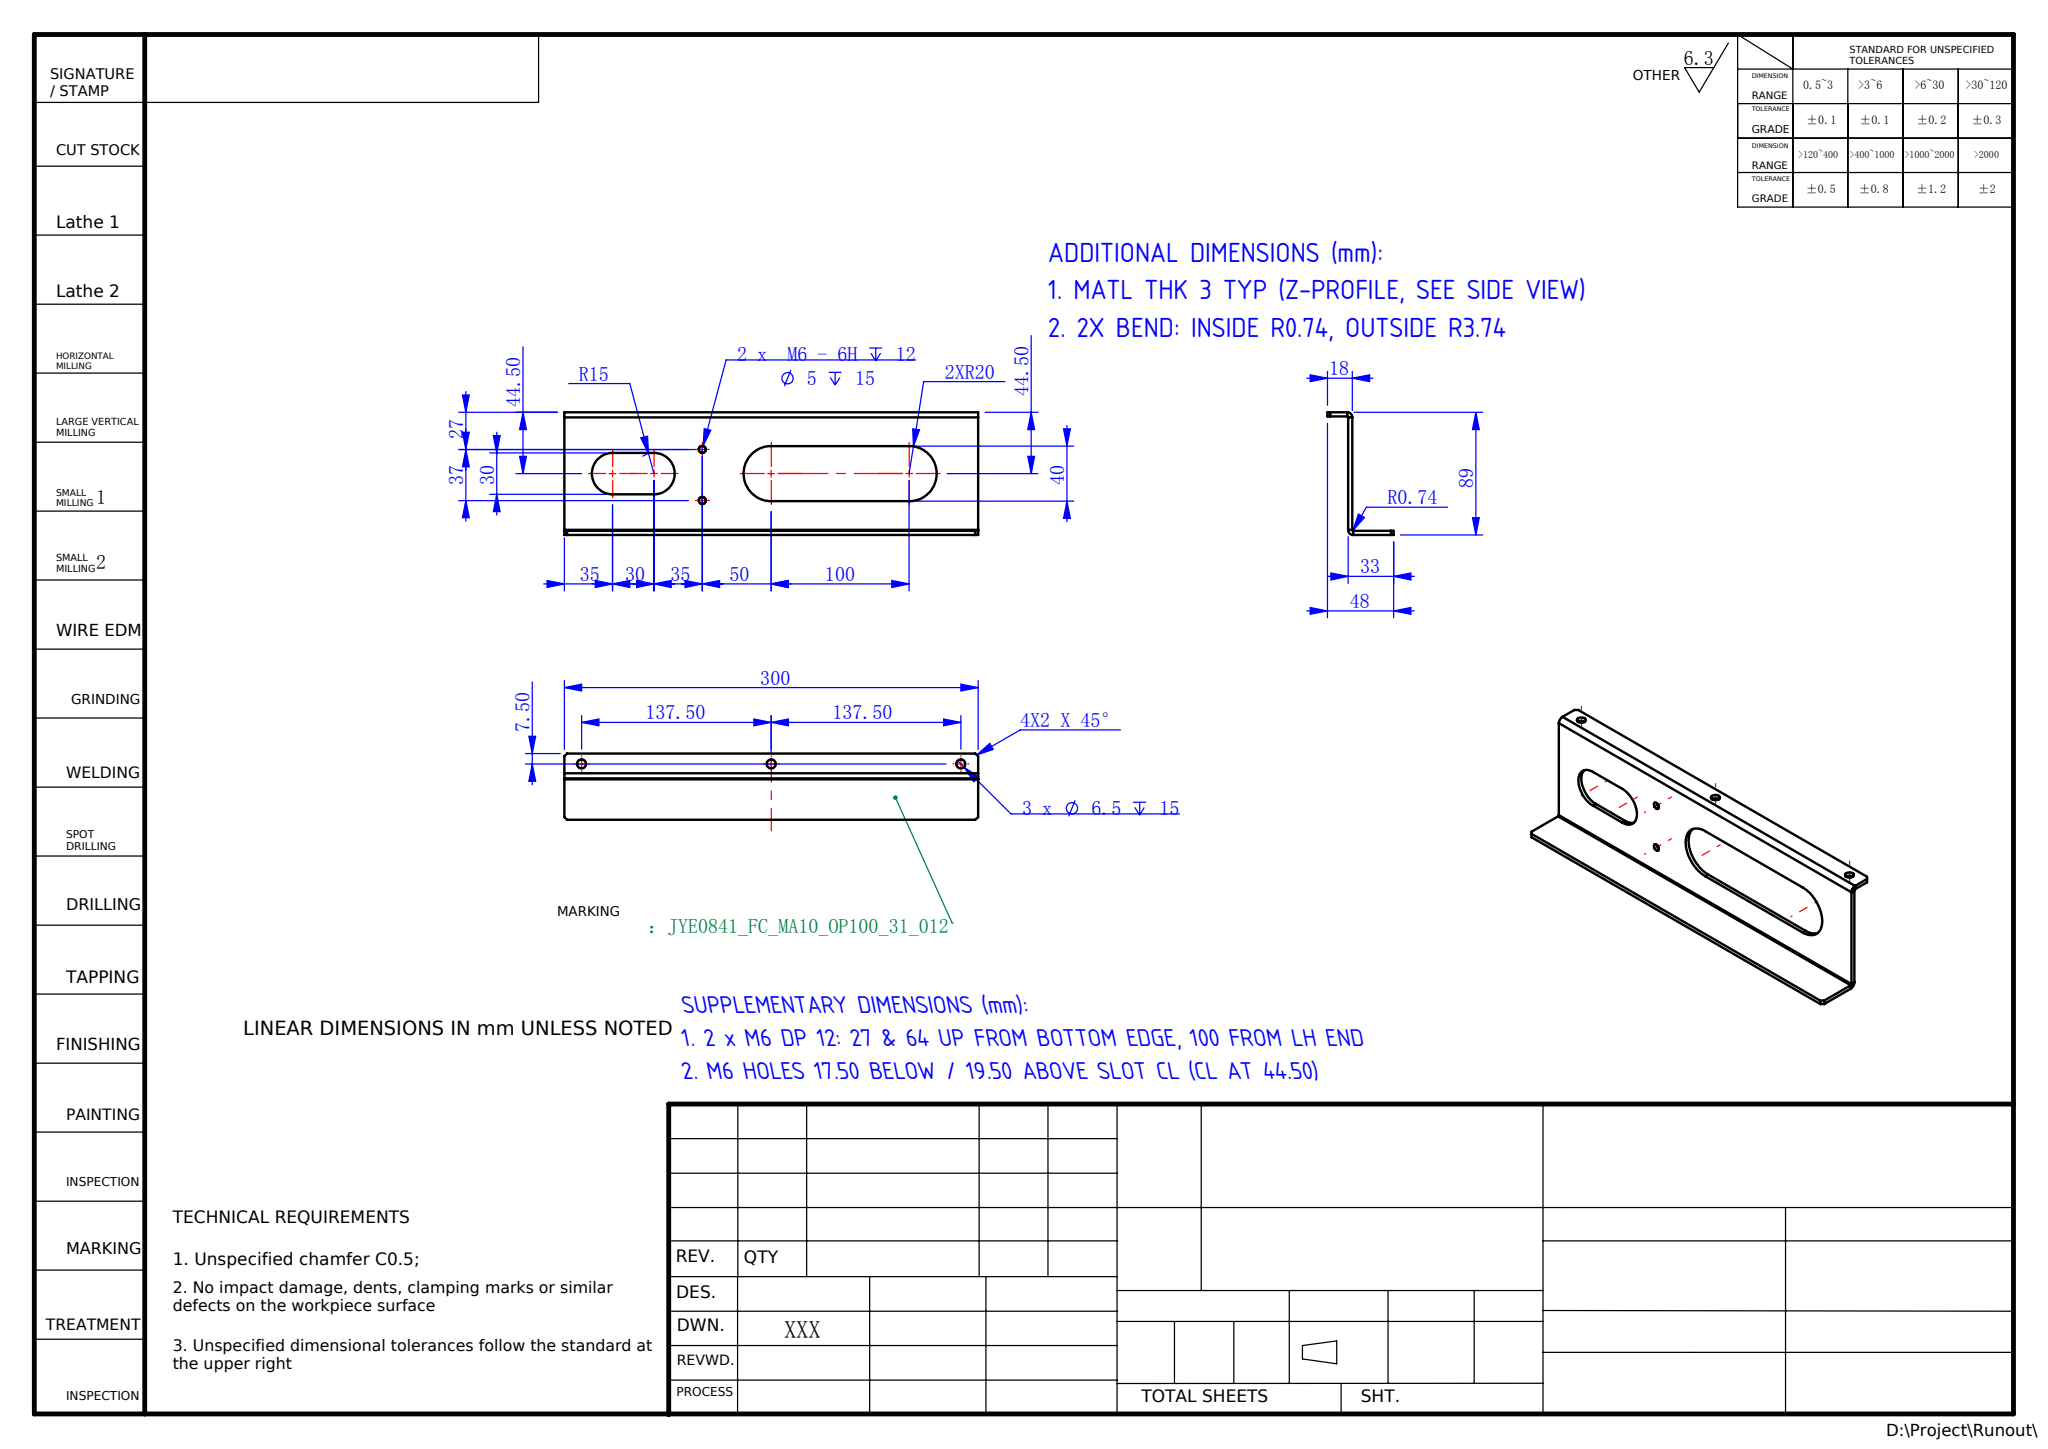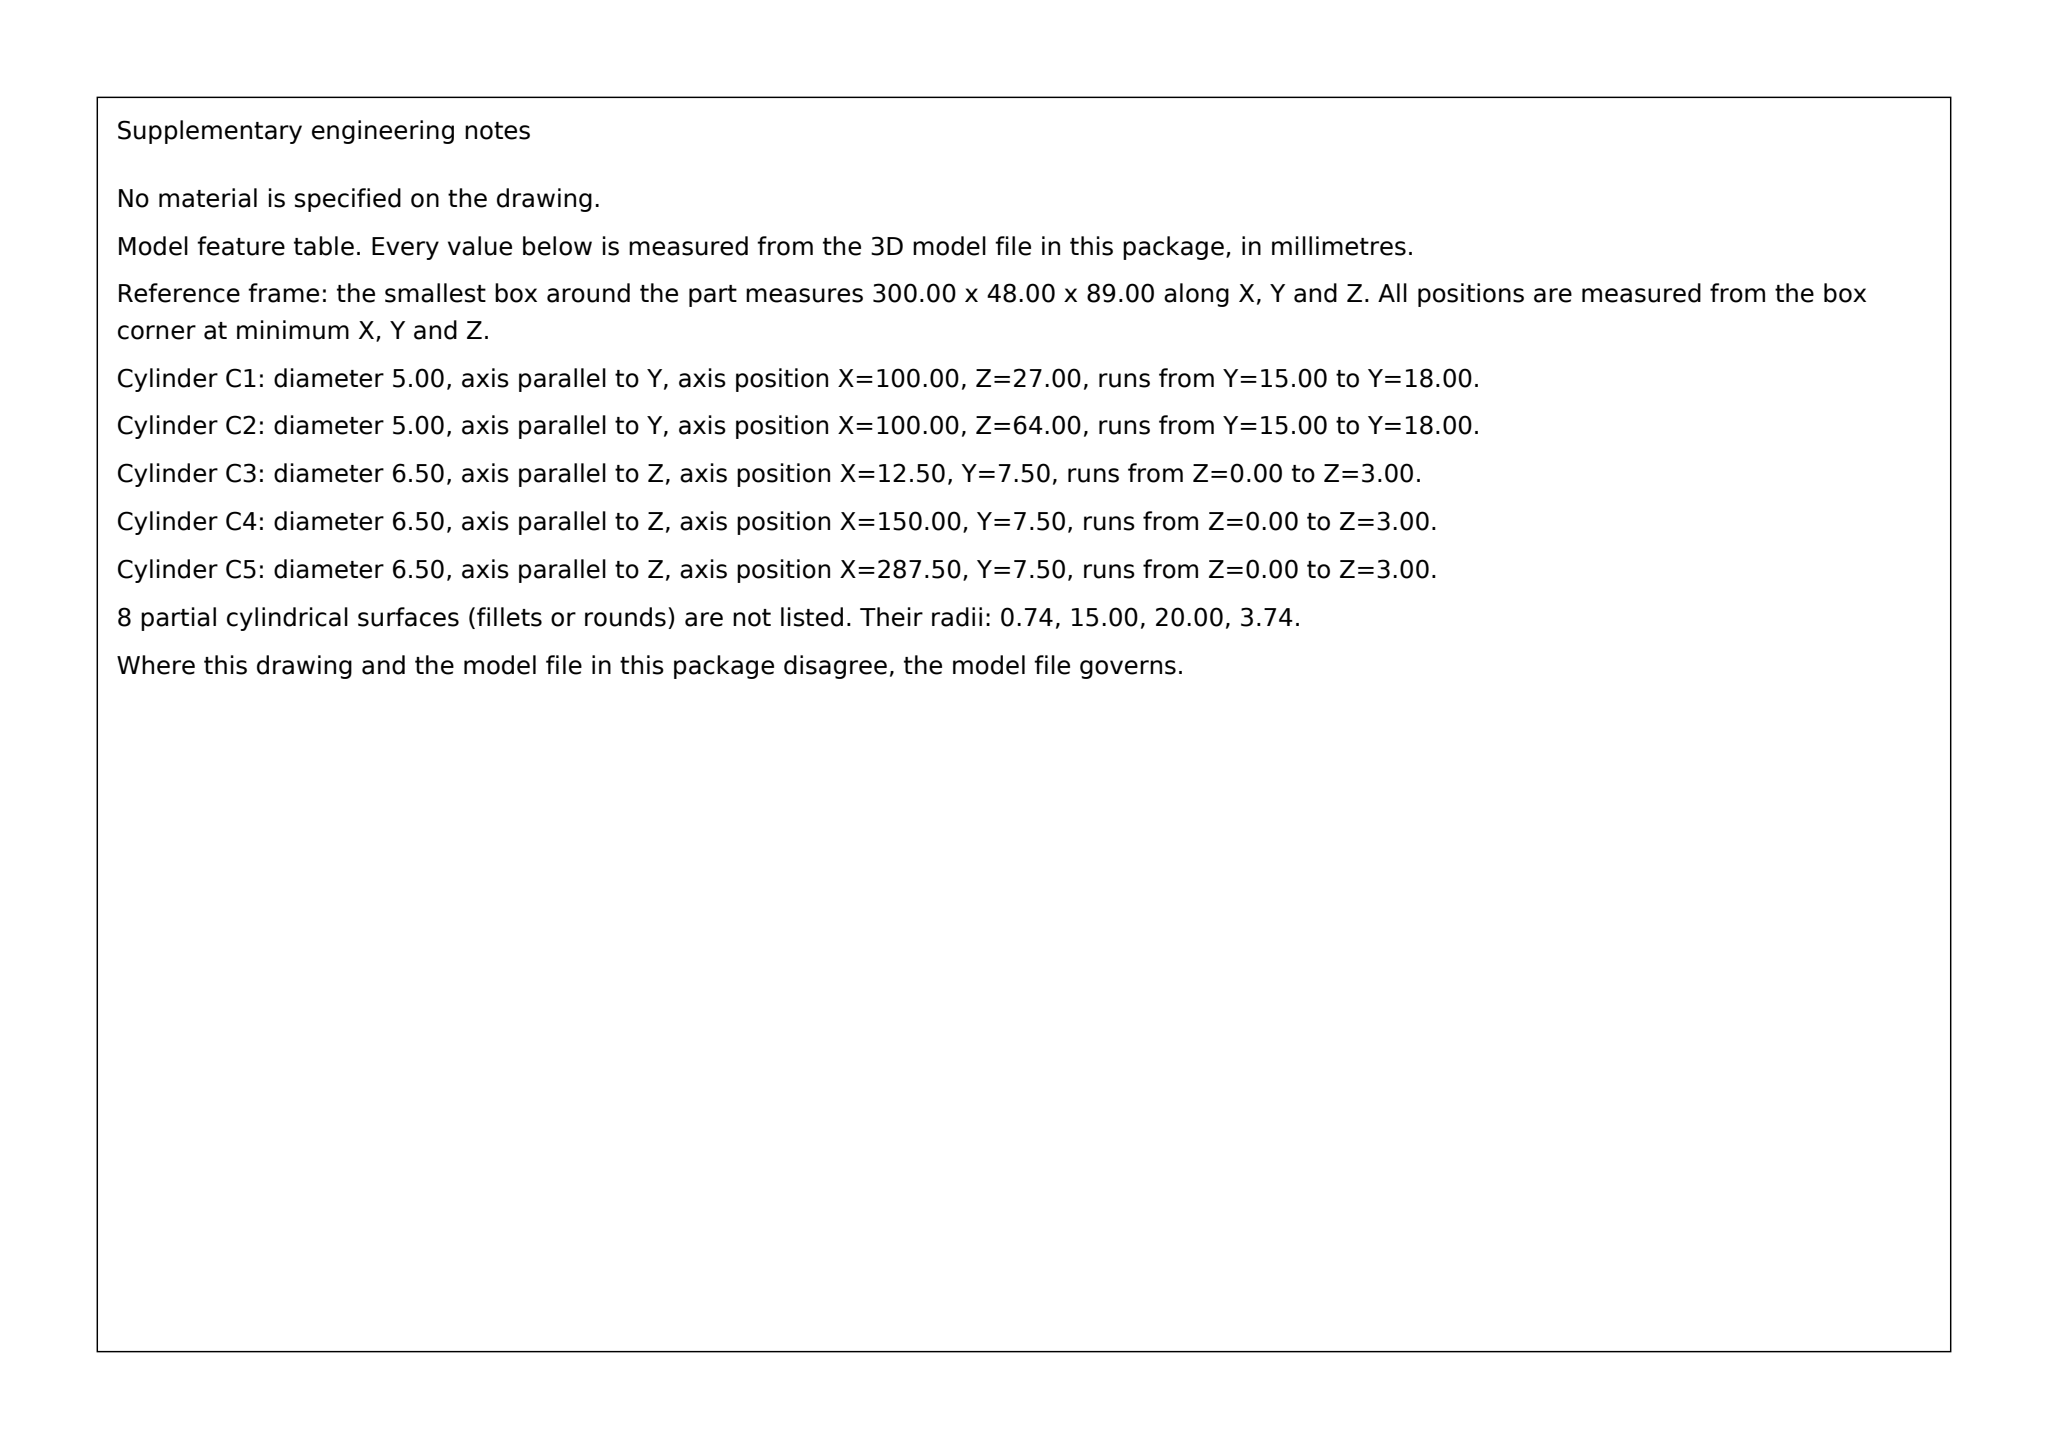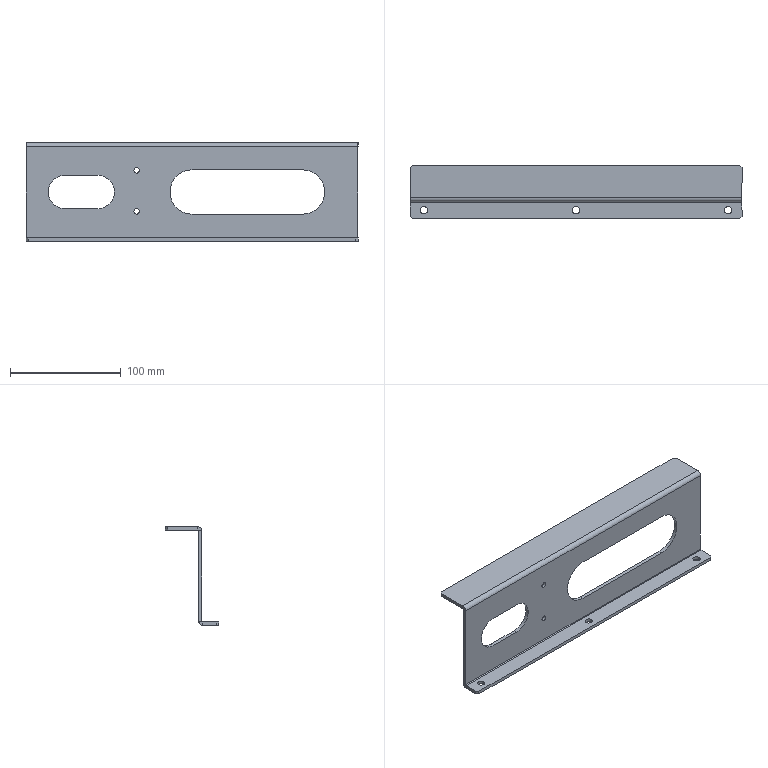Part | SolidWorks | mm | 1 solid | 44 faces | box 300 x 48 x 89 mm | volume 97841 mm3 | plane 26 | cylinder 18 | commonest cylinder face diameters 6.5 x6 5 x4 7.473 x2 1.473 x2 40 x2 30 x2